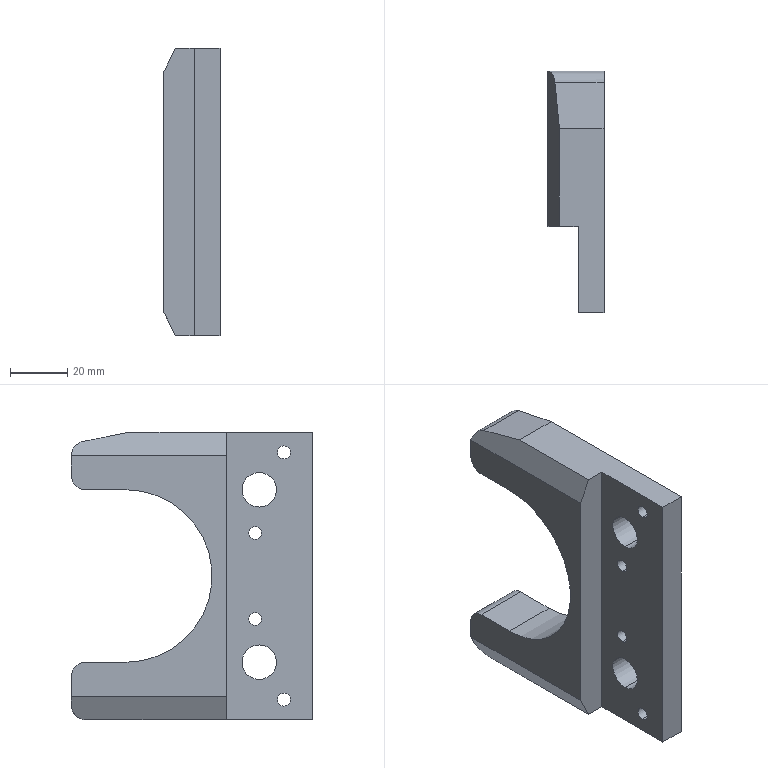Component | SolidWorks | QX1-17-V-BracketSidePlate-2 | 1 solid | 39 faces | box 19.5 x 84 x 100 mm | volume 76956 mm3 | cylinder 17 | plane 14 | cone 8 | commonest cylinder face diameters 4.5 x8 12 x4 10 x4 60 x1 | material PA Type 6
build123d program:
from build123d import *

# Parameters (mm, degrees)
SKETCH1_W                                            = 100
SKETCH1_H                                            = 60
BOSS_EXTRUDE1_DEPTH                                  = 15
SKETCH2_W                                            = 100
SKETCH2_H                                            = 30
CUT_EXTRUDE1_DEPTH                                   = 7
SKETCH4_R                                            = 6
CUT_EXTRUDE3_DEPTH                                   = 61.208
CONICAL_COUNTERSUNK_HOLE1_FOR_M4_HEXAGON_D           = 4.5
CONICAL_COUNTERSUNK_HOLE1_FOR_M4_HEXAGON_CSINK_D     = 9.18
CONICAL_COUNTERSUNK_HOLE1_FOR_M4_HEXAGON_CSINK_ANGLE = 90
MOVE_FACE1_BY                                        = 4.5
MOVE_FACE2_BY                                        = 30
SKETCH11_R                                           = 30
CUT_EXTRUDE5_DEPTH                                   = 81.5
SKETCH12_W                                           = 60
SKETCH12_H                                           = 25
CUT_EXTRUDE6_DEPTH                                   = 81.5
CHAMFER2_SIZE                                        = 8
CHAMFER2_SIZE2                                       = 4
CHAMFER3_SIZE                                        = 8
CHAMFER3_SIZE2                                       = 4
MOVE_FACE3_BY                                        = 6
MOVE_FACE3_2_BY                                      = 6
CHAMFER5_SIZE                                        = 4
CHAMFER5_SIZE2                                       = 20
FILLET5_R                                            = 5
MOVE_FACE4_BY                                        = 1


with BuildPart() as part:
    # Sketch1 → Boss-Extrude1 (new body)
    with BuildSketch(Plane.XY):
        Rectangle(SKETCH1_W, SKETCH1_H)
    extrude(amount=BOSS_EXTRUDE1_DEPTH)

    # Sketch2 → Cut-Extrude1 (cut)
    with BuildSketch(Plane(origin=(0, 0, 0), x_dir=(-1, 0, 0), z_dir=(0, 0, -1))):
        with Locations((0, 15)):
            Rectangle(SKETCH2_W, SKETCH2_H)
    extrude(amount=-CUT_EXTRUDE1_DEPTH, mode=Mode.SUBTRACT)

    # Sketch4 → Cut-Extrude3 (cut, through all)
    with BuildSketch(Plane.XY.offset(15)):
        with Locations((-30, 11.4)):
            Circle(SKETCH4_R)
        with Locations((30, 11.4)):
            Circle(SKETCH4_R)
    extrude(amount=-CUT_EXTRUDE3_DEPTH, mode=Mode.SUBTRACT)

    # Conical Countersunk Hole1 for M4 Hexagon (through all)
    with Locations(Plane.XY.offset(15)):
        with Locations((15, 10), (-15, 10), (43, 20), (-43, 20)):
            CounterSinkHole(CONICAL_COUNTERSUNK_HOLE1_FOR_M4_HEXAGON_D / 2, CONICAL_COUNTERSUNK_HOLE1_FOR_M4_HEXAGON_CSINK_D / 2, counter_sink_angle=CONICAL_COUNTERSUNK_HOLE1_FOR_M4_HEXAGON_CSINK_ANGLE)

    # Move Face1: a face moved outward by 4.5
    extrude(part.faces().sort_by_distance((0, -15, 0))[0], amount=MOVE_FACE1_BY, dir=(0, 0, -1))

    # Move Face2: a face moved outward by 30.0
    extrude(part.faces().sort_by_distance((0, -30, 5.25))[0], amount=MOVE_FACE2_BY, dir=(0, -1, 0))

    # Sketch11 → Cut-Extrude5 (cut, through all)
    with BuildSketch(Plane.XY.offset(15)):
        with Locations((0, -35)):
            Circle(SKETCH11_R)
    extrude(amount=-CUT_EXTRUDE5_DEPTH, mode=Mode.SUBTRACT)

    # Sketch12 → Cut-Extrude6 (cut, through all)
    with BuildSketch(Plane.XY.offset(15)):
        with Locations((0, -47.5)):
            Rectangle(SKETCH12_W, SKETCH12_H)
    extrude(amount=-CUT_EXTRUDE6_DEPTH, mode=Mode.SUBTRACT)

    # Chamfer2
    chamfer2_edges = [part.edges().sort_by_distance(p)[0] for p in [
        (-50, -30, -4.5),
    ]]
    chamfer2_side = [part.faces().sort_by_distance(p)[0] for p in [
        (0, -1.166, -4.5),
    ]]
    chamfer(chamfer2_edges, length=CHAMFER2_SIZE, length2=CHAMFER2_SIZE2, reference=chamfer2_side[0])

    # Chamfer3
    chamfer3_edges = [part.edges().sort_by_distance(p)[0] for p in [
        (50, -30, -4.5),
    ]]
    chamfer3_side = [part.faces().sort_by_distance(p)[0] for p in [
        (4, -1.098, -4.5),
    ]]
    chamfer(chamfer3_edges, length=CHAMFER3_SIZE, length2=CHAMFER3_SIZE2, reference=chamfer3_side[0])

    # Move Face3: a face moved inward by 6.0
    extrude(part.faces().sort_by_distance((-39.686, -60, 5.61))[0], amount=MOVE_FACE3_BY, dir=(0, 1, 0), mode=Mode.SUBTRACT)

    # Move Face3 2: a face moved inward by 6.0
    extrude(part.faces().sort_by_distance((39.686, -60, 5.61))[0], amount=MOVE_FACE3_2_BY, dir=(0, 1, 0), mode=Mode.SUBTRACT)

    # Chamfer5
    chamfer5_edges = [part.edges().sort_by_distance(p)[0] for p in [
        (50, -54, 7.25),
    ]]
    chamfer5_side = [part.faces().sort_by_distance(p)[0] for p in [
        (39.686, -54, 5.61),
    ]]
    chamfer(chamfer5_edges, length=CHAMFER5_SIZE, length2=CHAMFER5_SIZE2, reference=chamfer5_side[0])

    # Fillet5
    fillet5_edges = [part.edges().sort_by_distance(p)[0] for p in [
        (-50, -54, 7.25),
        (-30, -54, 5.25),
        (30, -54, 5.25),
        (46, -54, 6.25),
    ]]
    fillet(fillet5_edges, radius=FILLET5_R)

    # Move Face4: a face moved outward by 1.0
    extrude(part.faces().sort_by_distance((0, 15.3, 7))[0], amount=MOVE_FACE4_BY, dir=(0, 0, -1))


solid = part.part

# Placed as in the assembly
solid = solid.moved(Location((17, 102, 0), (180, 90, 0)))